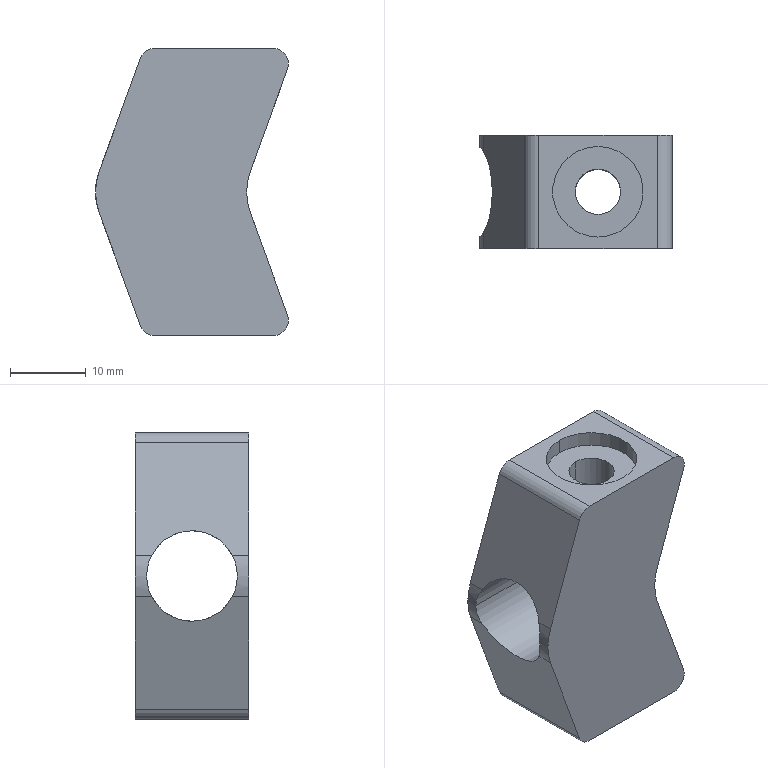Component | SolidWorks | MuzzleBrake-1 | 1 solid | 28 faces | box 25.55 x 15 x 38 mm | volume 7989 mm3 | cylinder 18 | plane 10 | commonest cylinder face diameters 12 x6 6 x4 16 x4 4 x4
build123d program:
from build123d import *

# Parameters (mm, degrees)
BOSS_EXTRUDE1_DEPTH = 15
SKETCH2_R           = 6
CUT_EXTRUDE1_DEPTH  = 32


with BuildPart() as part:
    # Sketch1 → Boss-Extrude1 (new body)
    with BuildSketch(Plane.XY):
        with BuildLine():
            Line((-19, -8.316), (-19, -24.066))
            ThreePointArc((-19, -24.066), (-18.147, -25.704), (-16.316, -25.945))
            Line((-16.316, -25.945), (-2.736, -21.002))
            ThreePointArc((-2.736, -21.002), (0, -20.52), (2.736, -21.002))
            Line((2.736, -21.002), (16.316, -25.945))
            ThreePointArc((16.316, -25.945), (18.147, -25.704), (19, -24.066))
            Line((19, -24.066), (19, -8.316))
            ThreePointArc((19, -8.316), (18.638, -7.169), (17.684, -6.436))
            Line((17.684, -6.436), (2.736, -0.9959))
            ThreePointArc((2.736, -0.9959), (0, -0.5134), (-2.736, -0.9959))
            Line((-2.736, -0.9959), (-17.684, -6.436))
            ThreePointArc((-17.684, -6.436), (-18.638, -7.169), (-19, -8.316))
        make_face()
    extrude(amount=BOSS_EXTRUDE1_DEPTH)

    # Sketch2 → Cut-Extrude1 (cut)
    with BuildSketch(Plane(origin=(0, 0, 0), x_dir=(1, 0, 0), z_dir=(0, 1, 0))):
        with Locations(Location((0, -7.5, 0), (0, 0, 242.869))):
            Circle(SKETCH2_R)
    extrude(amount=-CUT_EXTRUDE1_DEPTH, mode=Mode.SUBTRACT)

    # Sketch6 → Cylindrical Countersunk Hole for M6 Hex (revolve, cut)
    with BuildSketch(Plane(origin=(19, -16.191, 7.5), x_dir=(0, 0, -1), z_dir=(0, 1, 0))):
        Polygon((0, 0), (0, 16.803), (3, 15), (3, 2), (6, 2), (6, 0), align=None)
    cylindrical_countersunk_hole_for_m6_hex = revolve(axis=Axis((25.35, -16.191, 7.5), (-1, 0, 0)), mode=Mode.SUBTRACT)

    # Mirror1: Cylindrical Countersunk Hole for M6 Hex across plane
    add(cylindrical_countersunk_hole_for_m6_hex.mirror(Plane(origin=(0, 0, 0), x_dir=(0, 0, 1), z_dir=(1, 0, 0))), mode=Mode.SUBTRACT)


solid = part.part

# Placed as in the assembly
solid = solid.moved(Location((-417.008, 41.983, 1009), (90, 0, 90)))